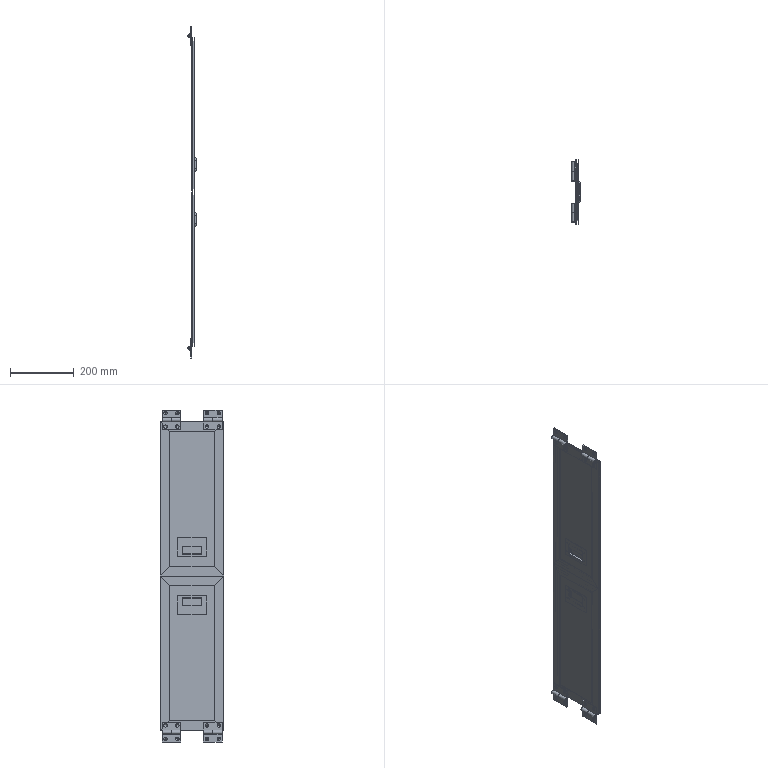Component | SolidWorks | 30-01A-1_AluminumAlloyDoorAcrylicPlate(UpperSmallDoor)-1 | 24 solids | 482 faces | volume 1107230 mm3 | plane 282 | cylinder 152 | cone 32 | torus 16 | commonest cylinder face diameters 5.5 x32 2 x32 10 x32 16 x16 4.5 x16 6 x8 12 x8 4 x8